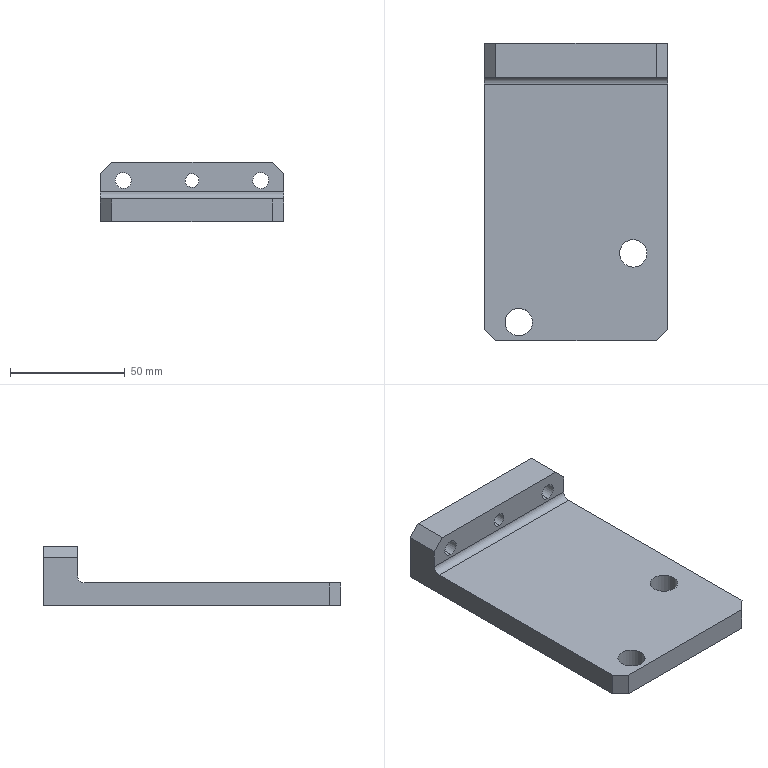CAM job | Mastercam | mm | 16 operations | part box 80 x 130 x 26
1. Facing | 24 - 100 平铣刀
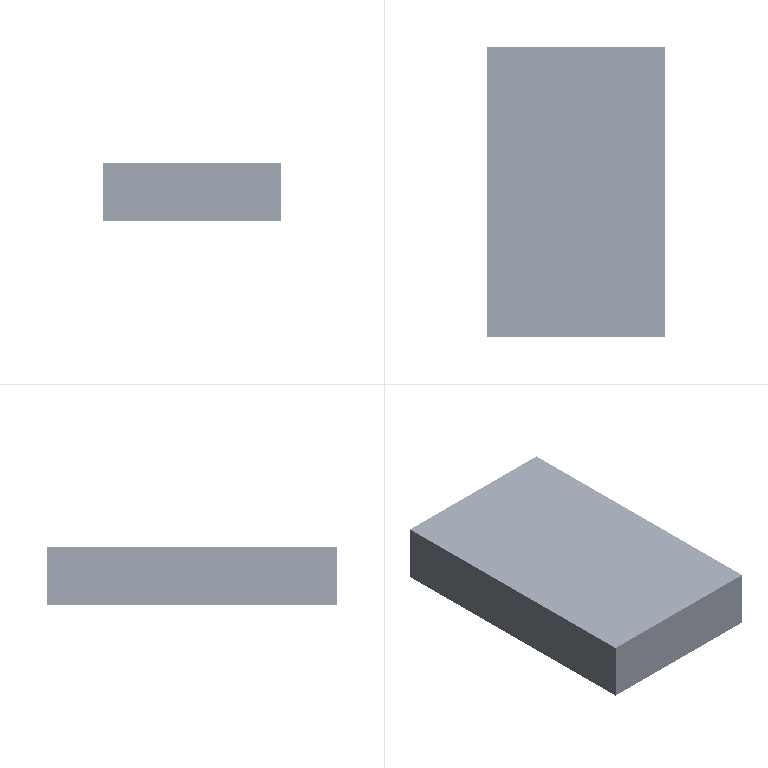2. Contour (Ramp) | 9 - 10 平铣刀
3. 3D High Speed (Area roughing) | 9 - 10 平铣刀
4. Contour (2D) | 10 - 10 平铣刀
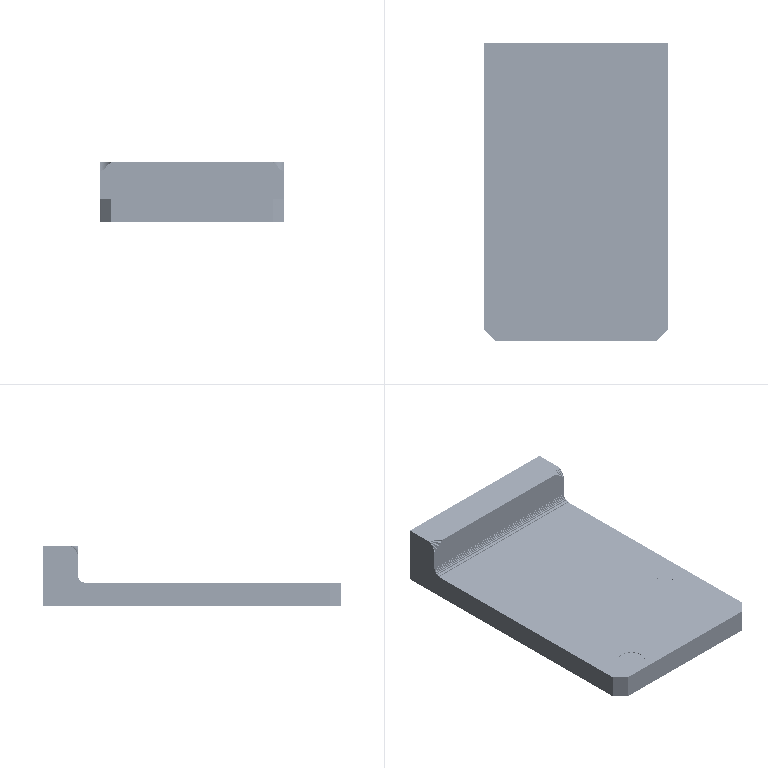5. Contour (2D) | 10 - 10 平铣刀
6. Facing | 10 - 10 平铣刀
7. Contour (2D) | 10 - 10 平铣刀
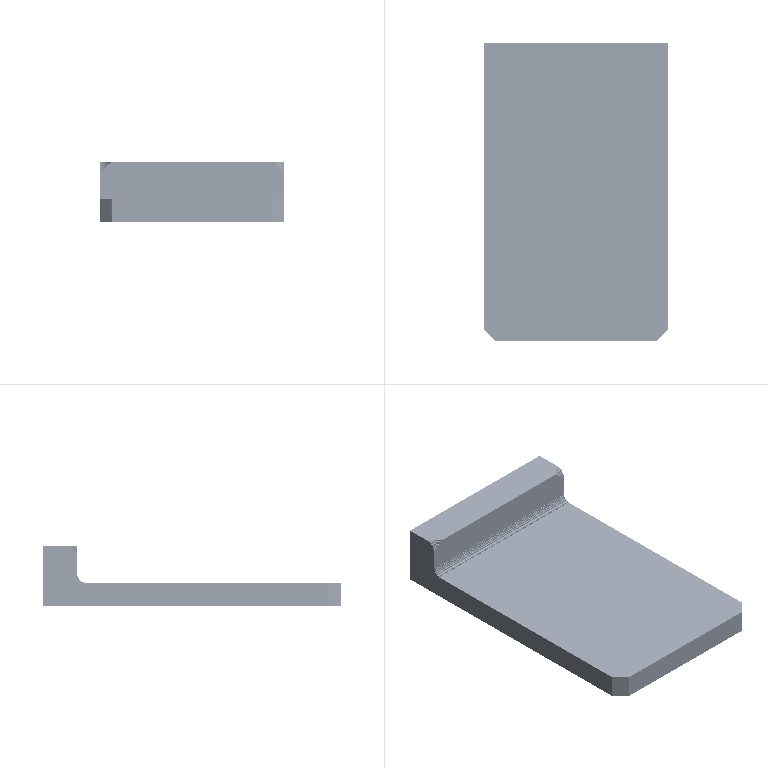8. Contour (2D) | 17 - 6 球刀/圆鼻铣刀
9. Surface Finish Flowline | 17 - 6 球刀/圆鼻铣刀
10. Contour (Ramp) | 6 - 6 平铣刀
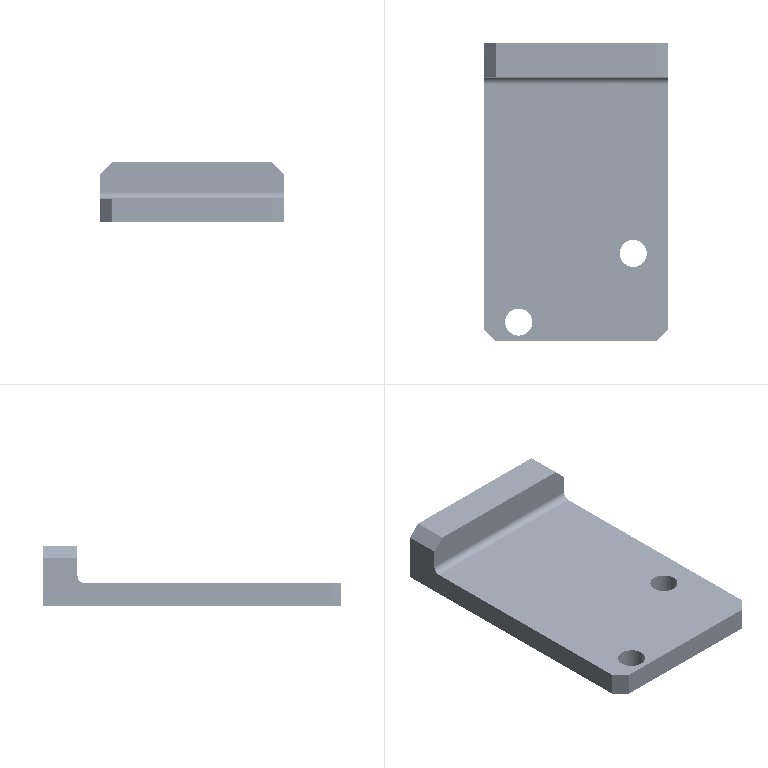11. Deburr 5-axis | 17 - 6 球刀/圆鼻铣刀
12. Contour (Ramp) | 6 - 6 平铣刀
13. Facing | 9 - 10 平铣刀
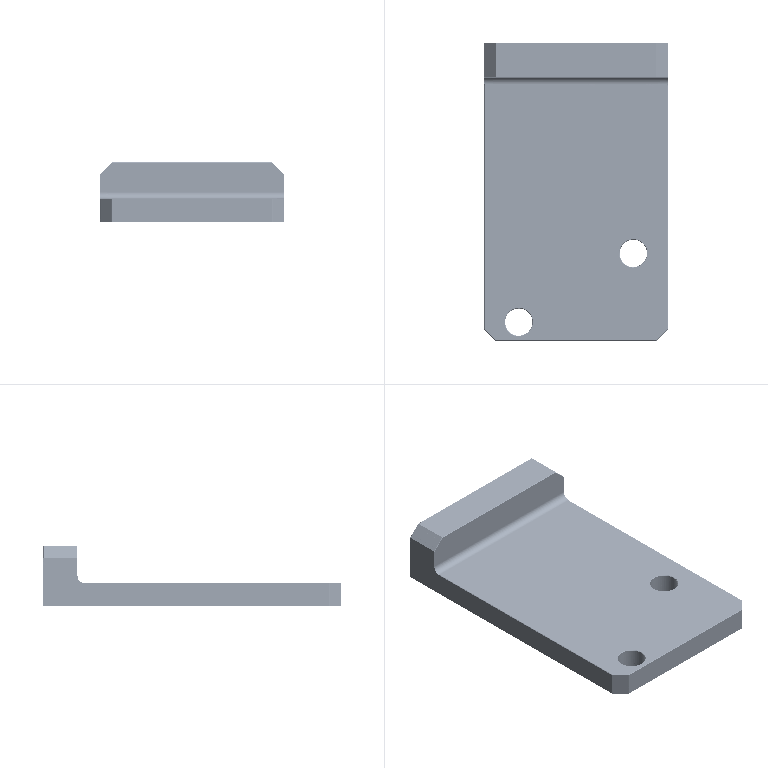14. Facing | 24 - 100 平铣刀
15. Contour (2D chamfer) | 5 - 4 倒角刀
16. Drill/Counterbore | 5 - 4 倒角刀